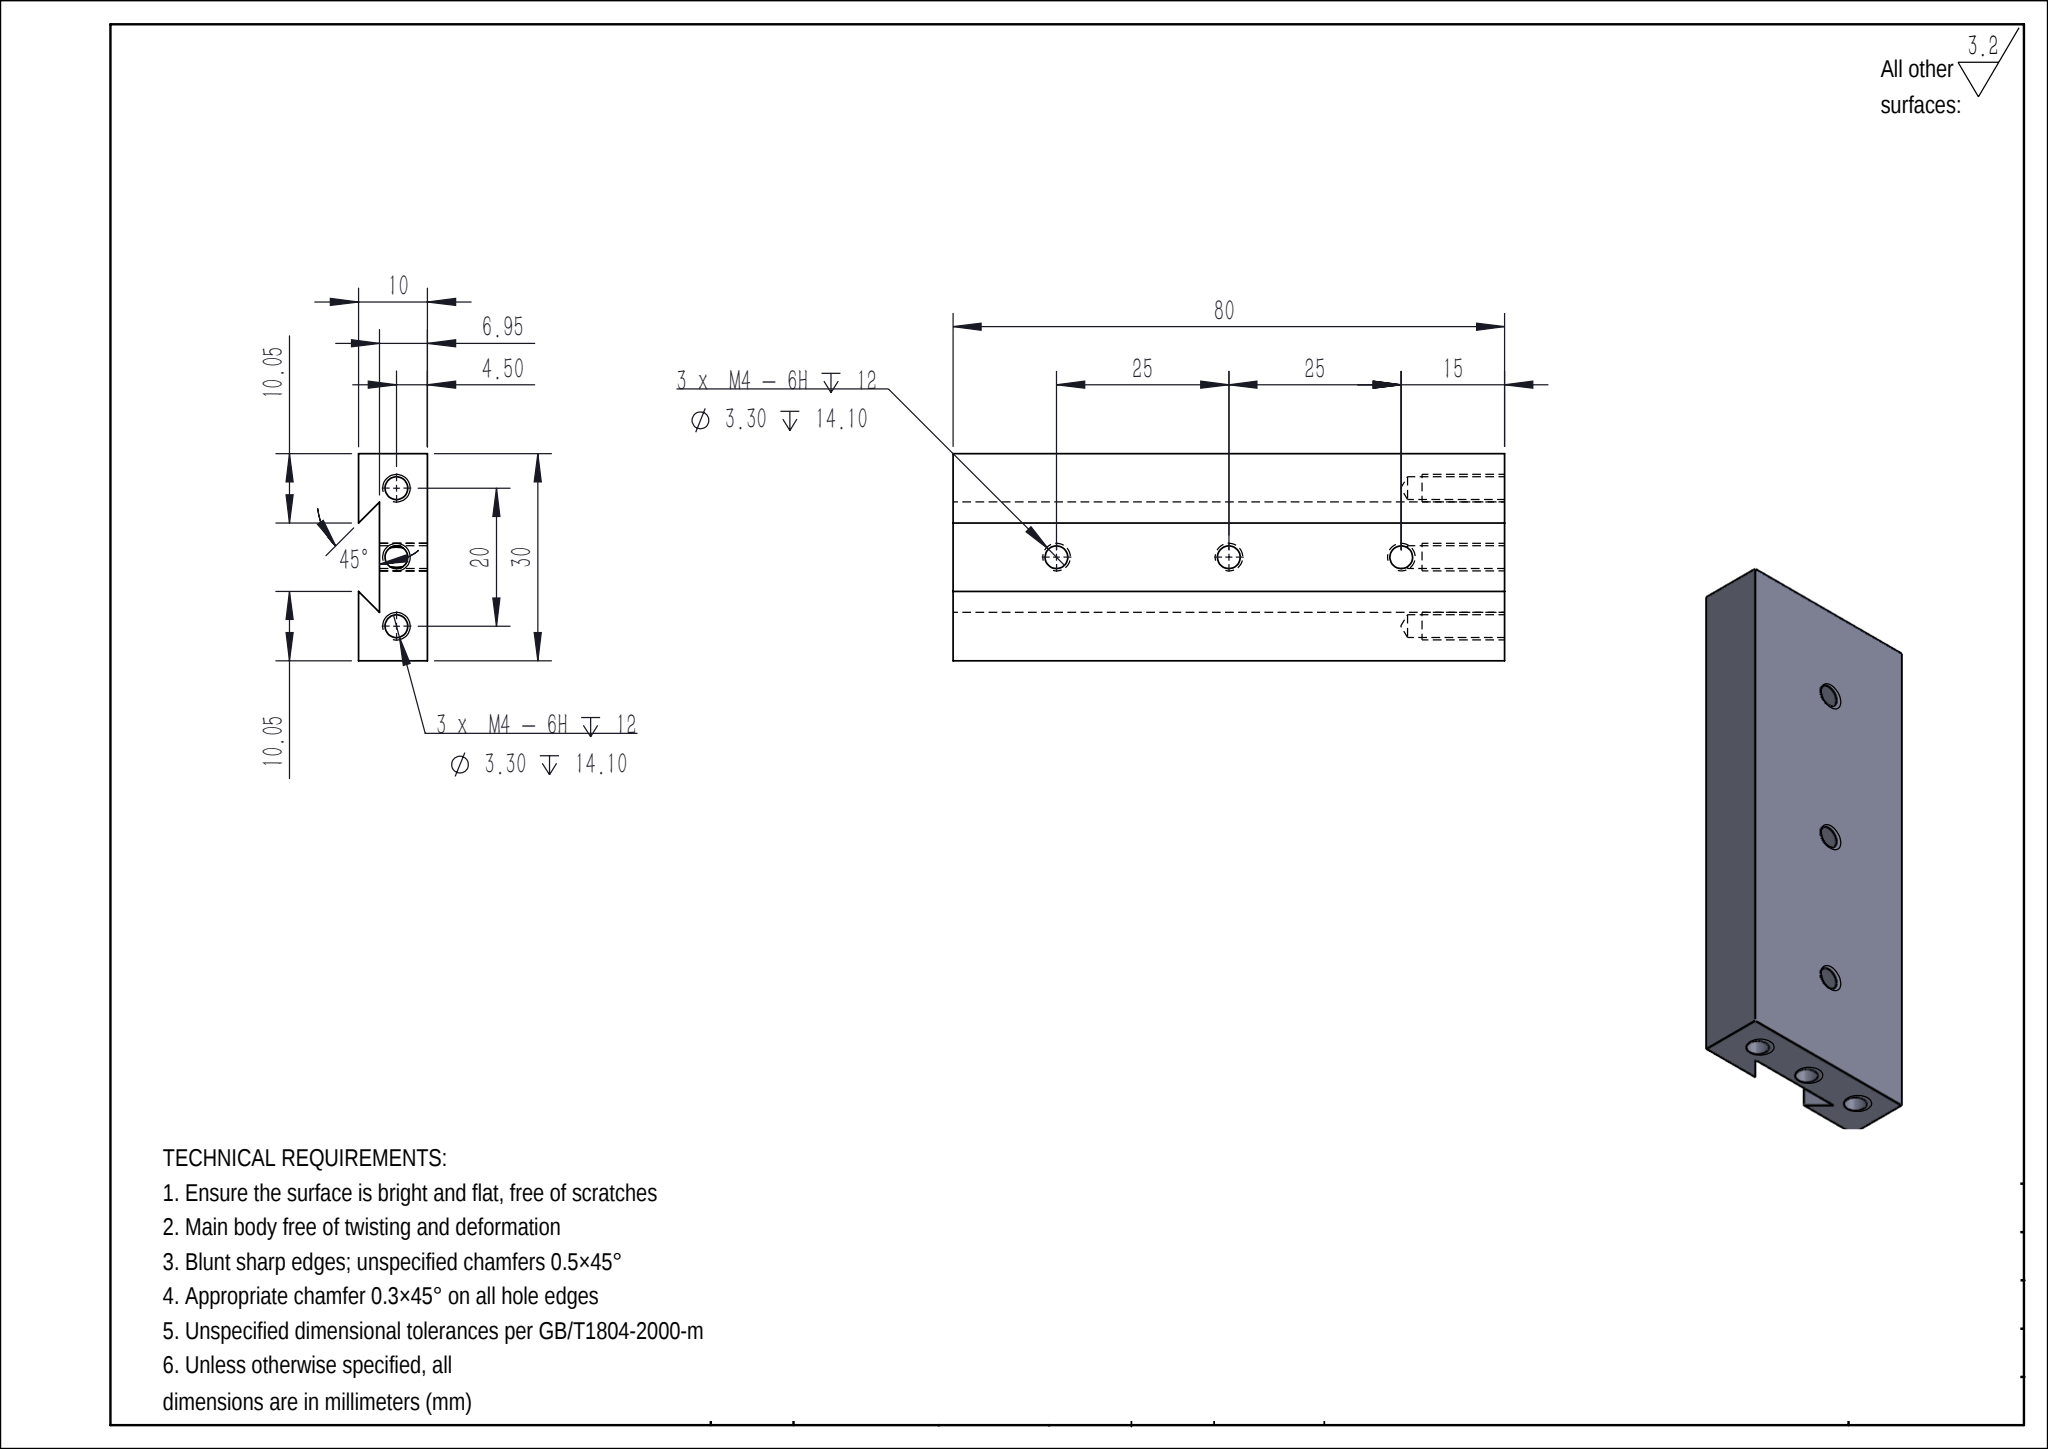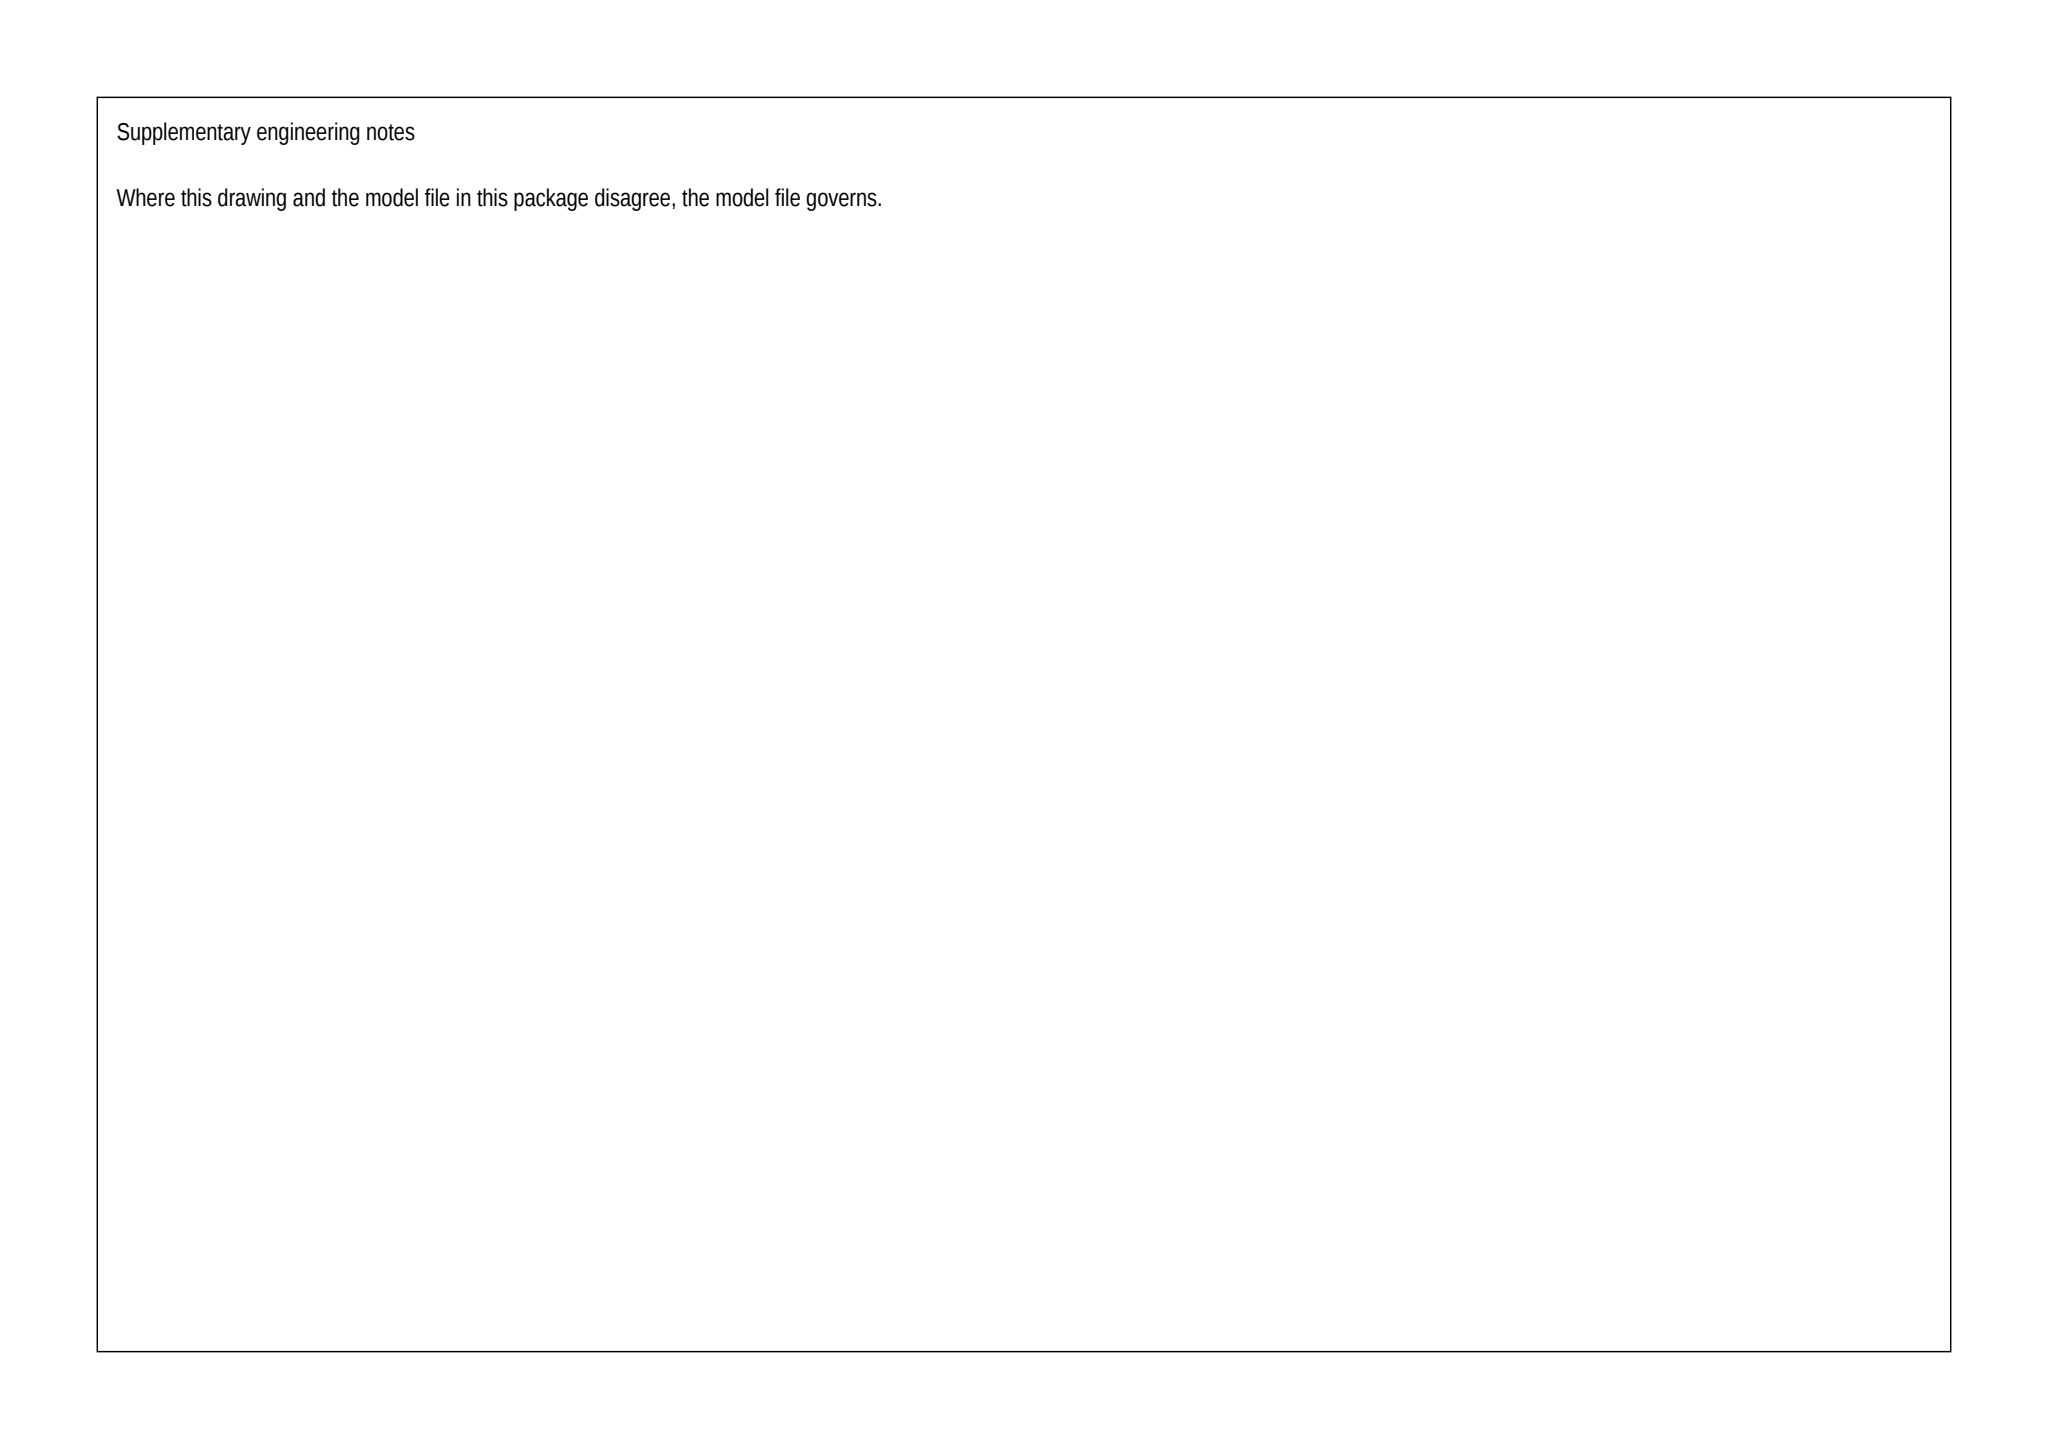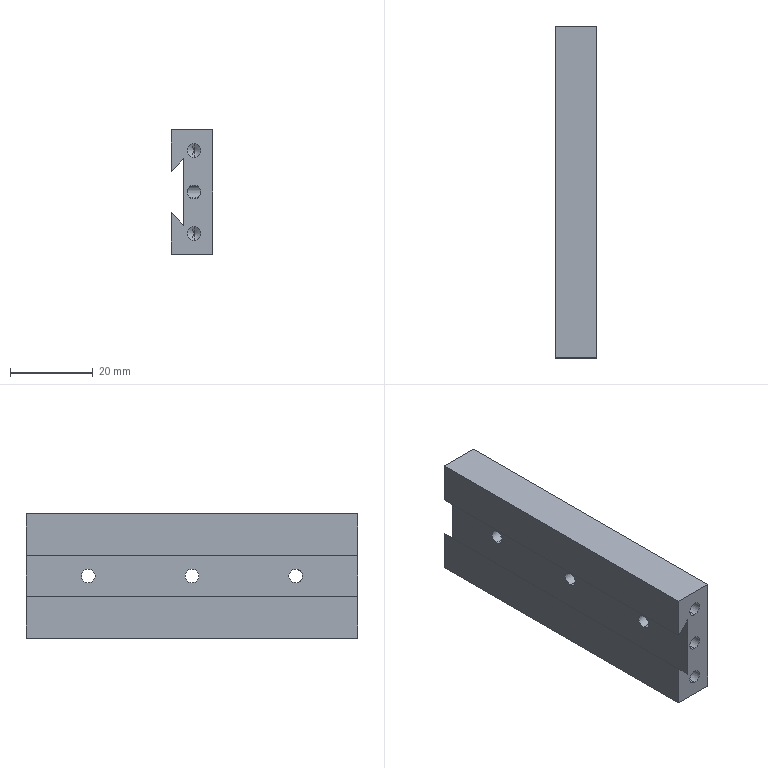Part | SolidWorks | mm | 1 solid | 29 faces | box 10 x 80 x 30 mm | volume 20299 mm3 | cylinder 12 | plane 10 | cone 7 | commonest cylinder face diameters 3.3 x12
build123d program:
from build123d import *

# Parameters (mm, degrees)
SKETCH1_W             = 10
SKETCH1_H             = 80
EXTRUDE_THIN1_DEPTH   = 30
CUT_EXTRUDE1_DEPTH    = 100
M4_TAPPED_HOLE1_D     = 3.3
M4_TAPPED_HOLE1_DEPTH = 14.1
M4_TAPPED_HOLE1_TIP   = 0.9914
M4_TAPPED_HOLE2_D     = 3.3
M4_TAPPED_HOLE2_DEPTH = 14.1
M4_TAPPED_HOLE2_TIP   = 0.9914


with BuildPart() as part:
    # Sketch1 → Extrude-Thin1 (new body)
    with BuildSketch(Plane.XY):
        with Locations((5, 40)):
            Rectangle(SKETCH1_W, SKETCH1_H)
    extrude(amount=EXTRUDE_THIN1_DEPTH)

    # Sketch2 → Cut-Extrude1 (cut)
    with BuildSketch(Plane(origin=(0, 80, 0), x_dir=(1, 0, 0), z_dir=(0, 1, 0))):
        Polygon((0, -10.05), (0, -19.95), (3.05, -23), (3.05, -7), align=None)
    extrude(amount=-CUT_EXTRUDE1_DEPTH, mode=Mode.SUBTRACT)

    # M4 Tapped Hole1
    with Locations(Plane(origin=(0, 0, 0), x_dir=(-1, 0, 0), z_dir=(0, -1, 0))):
        with Locations((-5.5, -5), (-5.5, -25), (-5.5, -15)):
            Hole(M4_TAPPED_HOLE1_D / 2, depth=M4_TAPPED_HOLE1_DEPTH)
            with Locations((0, 0, -(M4_TAPPED_HOLE1_DEPTH + M4_TAPPED_HOLE1_TIP / 2))):  # 118° drill point
                Cone(0, M4_TAPPED_HOLE1_D / 2, M4_TAPPED_HOLE1_TIP, mode=Mode.SUBTRACT)

    # M4 Tapped Hole2
    with Locations(Plane(origin=(10, 0, 0), x_dir=(0, 0, -1), z_dir=(1, 0, 0))):
        with Locations((-15, 40), (-15, 15), (-15, 65)):
            Hole(M4_TAPPED_HOLE2_D / 2, depth=M4_TAPPED_HOLE2_DEPTH)
            with Locations((0, 0, -(M4_TAPPED_HOLE2_DEPTH + M4_TAPPED_HOLE2_TIP / 2))):  # 118° drill point
                Cone(0, M4_TAPPED_HOLE2_D / 2, M4_TAPPED_HOLE2_TIP, mode=Mode.SUBTRACT)


solid = part.part
STEP:
#1=CARTESIAN_POINT('',(3.05,40.,16.65));
#2=VERTEX_POINT('',#1);
#3=CARTESIAN_POINT('',(3.05,40.,13.35));
#4=VERTEX_POINT('',#3);
#5=CARTESIAN_POINT('',(3.05,40.,15.));
#6=DIRECTION('',(1.,0.,0.));
#7=DIRECTION('',(0.,0.,-1.));
#8=AXIS2_PLACEMENT_3D('',#5,#6,#7);
#9=CIRCLE('',#8,1.65);
#10=EDGE_CURVE('',#2,#4,#9,.T.);
#11=ORIENTED_EDGE('',*,*,#10,.F.);
#12=CARTESIAN_POINT('',(10.,40.,16.65));
#13=VERTEX_POINT('',#12);
#14=CARTESIAN_POINT('',(10.,40.,16.65));
#15=DIRECTION('',(1.,0.,0.));
#16=VECTOR('',#15,1000.);
#17=LINE('',#14,#16);
#18=EDGE_CURVE('',#2,#13,#17,.T.);
#19=ORIENTED_EDGE('',*,*,#18,.T.);
#20=CARTESIAN_POINT('',(10.,40.,13.35));
#21=VERTEX_POINT('',#20);
#22=CARTESIAN_POINT('',(10.,40.,15.));
#23=DIRECTION('',(1.,0.,0.));
#24=DIRECTION('',(0.,0.,-1.));
#25=AXIS2_PLACEMENT_3D('',#22,#23,#24);
#26=CIRCLE('',#25,1.65);
#27=EDGE_CURVE('',#13,#21,#26,.T.);
#28=ORIENTED_EDGE('',*,*,#27,.T.);
#29=CARTESIAN_POINT('',(10.,40.,13.35));
#30=DIRECTION('',(1.,0.,0.));
#31=VECTOR('',#30,1000.);
#32=LINE('',#29,#31);
#33=EDGE_CURVE('',#4,#21,#32,.T.);
#34=ORIENTED_EDGE('',*,*,#33,.F.);
#35=EDGE_LOOP('',(#11,#19,#28,#34));
#36=FACE_OUTER_BOUND('',#35,.T.);
#37=CARTESIAN_POINT('',(10.,40.,15.));
#38=DIRECTION('',(1.,0.,0.));
#39=DIRECTION('',(0.,0.,-1.));
#40=AXIS2_PLACEMENT_3D('',#37,#38,#39);
#41=CYLINDRICAL_SURFACE('',#40,1.65);
#42=ADVANCED_FACE('',(#36),#41,.F.);
#43=CARTESIAN_POINT('',(6.4,14.1,16.383));
#44=VERTEX_POINT('',#43);
#45=CARTESIAN_POINT('',(6.4,14.1,13.617));
#46=VERTEX_POINT('',#45);
#47=CARTESIAN_POINT('',(6.4,14.1,16.383));
#48=CARTESIAN_POINT('',(7.509,12.991,15.661));
#49=CARTESIAN_POINT('',(7.509,12.991,14.339));
#50=CARTESIAN_POINT('',(6.4,14.1,13.617));
#51=(BOUNDED_CURVE()B_SPLINE_CURVE(3,(#47,#48,#49,#50),.UNSPECIFIED.,.F.,.F.)B_SPLINE_CURVE_WITH_KNOTS((4,4),(5.289,7.277),.UNSPECIFIED.)CURVE()GEOMETRIC_REPRESENTATION_ITEM()RATIONAL_B_SPLINE_CURVE((1.,0.697,0.697,1.))REPRESENTATION_ITEM(''));
#52=EDGE_CURVE('',#44,#46,#51,.T.);
#53=ORIENTED_EDGE('',*,*,#52,.F.);
#54=CARTESIAN_POINT('',(4.6,14.1,16.383));
#55=VERTEX_POINT('',#54);
#56=CARTESIAN_POINT('',(4.6,14.1,16.383));
#57=CARTESIAN_POINT('',(4.892,14.172,16.43));
#58=CARTESIAN_POINT('',(5.193,14.218,16.453));
#59=CARTESIAN_POINT('',(5.808,14.218,16.453));
#60=CARTESIAN_POINT('',(6.107,14.172,16.43));
#61=CARTESIAN_POINT('',(6.4,14.1,16.383));
#62=B_SPLINE_CURVE_WITH_KNOTS('',3,(#56,#57,#58,#59,#60,#61),.UNSPECIFIED.,.F.,.F.,(4,2,4),(0.0003713,0.001281,0.002191),.UNSPECIFIED.);
#63=EDGE_CURVE('',#55,#44,#62,.T.);
#64=ORIENTED_EDGE('',*,*,#63,.F.);
#65=CARTESIAN_POINT('',(4.6,14.1,13.617));
#66=VERTEX_POINT('',#65);
#67=CARTESIAN_POINT('',(4.6,14.1,13.617));
#68=CARTESIAN_POINT('',(3.491,12.991,14.339));
#69=CARTESIAN_POINT('',(3.491,12.991,15.661));
#70=CARTESIAN_POINT('',(4.6,14.1,16.383));
#71=(BOUNDED_CURVE()B_SPLINE_CURVE(3,(#67,#68,#69,#70),.UNSPECIFIED.,.F.,.F.)B_SPLINE_CURVE_WITH_KNOTS((4,4),(5.289,7.277),.UNSPECIFIED.)CURVE()GEOMETRIC_REPRESENTATION_ITEM()RATIONAL_B_SPLINE_CURVE((1.,0.697,0.697,1.))REPRESENTATION_ITEM(''));
#72=EDGE_CURVE('',#66,#55,#71,.T.);
#73=ORIENTED_EDGE('',*,*,#72,.F.);
#74=CARTESIAN_POINT('',(5.5,14.218,13.547));
#75=VERTEX_POINT('',#74);
#76=CARTESIAN_POINT('',(5.5,14.218,13.547));
#77=CARTESIAN_POINT('',(5.192,14.218,13.547));
#78=CARTESIAN_POINT('',(4.893,14.172,13.57));
#79=CARTESIAN_POINT('',(4.6,14.1,13.617));
#80=B_SPLINE_CURVE_WITH_KNOTS('',3,(#76,#77,#78,#79),.UNSPECIFIED.,.F.,.F.,(4,4),(0.00128,0.002191),.UNSPECIFIED.);
#81=EDGE_CURVE('',#75,#66,#80,.T.);
#82=ORIENTED_EDGE('',*,*,#81,.F.);
#83=CARTESIAN_POINT('',(6.4,14.1,13.617));
#84=CARTESIAN_POINT('',(6.109,14.172,13.57));
#85=CARTESIAN_POINT('',(5.807,14.218,13.547));
#86=CARTESIAN_POINT('',(5.5,14.218,13.547));
#87=B_SPLINE_CURVE_WITH_KNOTS('',3,(#83,#84,#85,#86),.UNSPECIFIED.,.F.,.F.,(4,4),(0.0003713,0.00128),.UNSPECIFIED.);
#88=EDGE_CURVE('',#46,#75,#87,.T.);
#89=ORIENTED_EDGE('',*,*,#88,.F.);
#90=EDGE_LOOP('',(#53,#64,#73,#82,#89));
#91=FACE_BOUND('',#90,.T.);
#92=CARTESIAN_POINT('',(3.05,15.,16.65));
#93=VERTEX_POINT('',#92);
#94=CARTESIAN_POINT('',(3.05,15.,13.35));
#95=VERTEX_POINT('',#94);
#96=CARTESIAN_POINT('',(3.05,15.,15.));
#97=DIRECTION('',(1.,0.,0.));
#98=DIRECTION('',(0.,0.,-1.));
#99=AXIS2_PLACEMENT_3D('',#96,#97,#98);
#100=CIRCLE('',#99,1.65);
#101=EDGE_CURVE('',#93,#95,#100,.T.);
#102=ORIENTED_EDGE('',*,*,#101,.F.);
#103=CARTESIAN_POINT('',(10.,15.,16.65));
#104=VERTEX_POINT('',#103);
#105=CARTESIAN_POINT('',(10.,15.,16.65));
#106=DIRECTION('',(1.,0.,0.));
#107=VECTOR('',#106,1000.);
#108=LINE('',#105,#107);
#109=EDGE_CURVE('',#93,#104,#108,.T.);
#110=ORIENTED_EDGE('',*,*,#109,.T.);
#111=CARTESIAN_POINT('',(10.,15.,13.35));
#112=VERTEX_POINT('',#111);
#113=CARTESIAN_POINT('',(10.,15.,15.));
#114=DIRECTION('',(1.,0.,0.));
#115=DIRECTION('',(0.,0.,-1.));
#116=AXIS2_PLACEMENT_3D('',#113,#114,#115);
#117=CIRCLE('',#116,1.65);
#118=EDGE_CURVE('',#104,#112,#117,.T.);
#119=ORIENTED_EDGE('',*,*,#118,.T.);
#120=CARTESIAN_POINT('',(10.,15.,13.35));
#121=DIRECTION('',(1.,0.,0.));
#122=VECTOR('',#121,1000.);
#123=LINE('',#120,#122);
#124=EDGE_CURVE('',#95,#112,#123,.T.);
#125=ORIENTED_EDGE('',*,*,#124,.F.);
#126=EDGE_LOOP('',(#102,#110,#119,#125));
#127=FACE_OUTER_BOUND('',#126,.T.);
#128=CARTESIAN_POINT('',(10.,15.,15.));
#129=DIRECTION('',(1.,0.,0.));
#130=DIRECTION('',(0.,0.,-1.));
#131=AXIS2_PLACEMENT_3D('',#128,#129,#130);
#132=CYLINDRICAL_SURFACE('',#131,1.65);
#133=ADVANCED_FACE('',(#91,#127),#132,.F.);
#134=CARTESIAN_POINT('',(3.05,65.,16.65));
#135=VERTEX_POINT('',#134);
#136=CARTESIAN_POINT('',(3.05,65.,13.35));
#137=VERTEX_POINT('',#136);
#138=CARTESIAN_POINT('',(3.05,65.,15.));
#139=DIRECTION('',(1.,0.,0.));
#140=DIRECTION('',(0.,0.,-1.));
#141=AXIS2_PLACEMENT_3D('',#138,#139,#140);
#142=CIRCLE('',#141,1.65);
#143=EDGE_CURVE('',#135,#137,#142,.T.);
#144=ORIENTED_EDGE('',*,*,#143,.F.);
#145=CARTESIAN_POINT('',(10.,65.,16.65));
#146=VERTEX_POINT('',#145);
#147=CARTESIAN_POINT('',(10.,65.,16.65));
#148=DIRECTION('',(1.,0.,0.));
#149=VECTOR('',#148,1000.);
#150=LINE('',#147,#149);
#151=EDGE_CURVE('',#135,#146,#150,.T.);
#152=ORIENTED_EDGE('',*,*,#151,.T.);
#153=CARTESIAN_POINT('',(10.,65.,13.35));
#154=VERTEX_POINT('',#153);
#155=CARTESIAN_POINT('',(10.,65.,15.));
#156=DIRECTION('',(1.,0.,0.));
#157=DIRECTION('',(0.,0.,-1.));
#158=AXIS2_PLACEMENT_3D('',#155,#156,#157);
#159=CIRCLE('',#158,1.65);
#160=EDGE_CURVE('',#146,#154,#159,.T.);
#161=ORIENTED_EDGE('',*,*,#160,.T.);
#162=CARTESIAN_POINT('',(10.,65.,13.35));
#163=DIRECTION('',(1.,0.,0.));
#164=VECTOR('',#163,1000.);
#165=LINE('',#162,#164);
#166=EDGE_CURVE('',#137,#154,#165,.T.);
#167=ORIENTED_EDGE('',*,*,#166,.F.);
#168=EDGE_LOOP('',(#144,#152,#161,#167));
#169=FACE_OUTER_BOUND('',#168,.T.);
#170=CARTESIAN_POINT('',(10.,65.,15.));
#171=DIRECTION('',(1.,0.,0.));
#172=DIRECTION('',(0.,0.,-1.));
#173=AXIS2_PLACEMENT_3D('',#170,#171,#172);
#174=CYLINDRICAL_SURFACE('',#173,1.65);
#175=ADVANCED_FACE('',(#169),#174,.F.);
#176=CARTESIAN_POINT('',(5.5,14.1,6.65));
#177=VERTEX_POINT('',#176);
#178=CARTESIAN_POINT('',(5.5,14.1,3.35));
#179=VERTEX_POINT('',#178);
#180=CARTESIAN_POINT('',(5.5,14.1,5.));
#181=DIRECTION('',(0.,-1.,0.));
#182=DIRECTION('',(0.,0.,-1.));
#183=AXIS2_PLACEMENT_3D('',#180,#181,#182);
#184=CIRCLE('',#183,1.65);
#185=EDGE_CURVE('',#177,#179,#184,.T.);
#186=ORIENTED_EDGE('',*,*,#185,.F.);
#187=CARTESIAN_POINT('',(5.5,-0.,6.65));
#188=VERTEX_POINT('',#187);
#189=CARTESIAN_POINT('',(5.5,0.,6.65));
#190=DIRECTION('',(0.,-1.,0.));
#191=VECTOR('',#190,1000.);
#192=LINE('',#189,#191);
#193=EDGE_CURVE('',#177,#188,#192,.T.);
#194=ORIENTED_EDGE('',*,*,#193,.T.);
#195=CARTESIAN_POINT('',(5.5,-0.,3.35));
#196=VERTEX_POINT('',#195);
#197=CARTESIAN_POINT('',(5.5,-0.,5.));
#198=DIRECTION('',(0.,-1.,0.));
#199=DIRECTION('',(0.,0.,-1.));
#200=AXIS2_PLACEMENT_3D('',#197,#198,#199);
#201=CIRCLE('',#200,1.65);
#202=EDGE_CURVE('',#188,#196,#201,.T.);
#203=ORIENTED_EDGE('',*,*,#202,.T.);
#204=CARTESIAN_POINT('',(5.5,0.,3.35));
#205=DIRECTION('',(0.,-1.,0.));
#206=VECTOR('',#205,1000.);
#207=LINE('',#204,#206);
#208=EDGE_CURVE('',#179,#196,#207,.T.);
#209=ORIENTED_EDGE('',*,*,#208,.F.);
#210=EDGE_LOOP('',(#186,#194,#203,#209));
#211=FACE_OUTER_BOUND('',#210,.T.);
#212=CARTESIAN_POINT('',(5.5,0.,5.));
#213=DIRECTION('',(0.,-1.,0.));
#214=DIRECTION('',(0.,0.,-1.));
#215=AXIS2_PLACEMENT_3D('',#212,#213,#214);
#216=CYLINDRICAL_SURFACE('',#215,1.65);
#217=ADVANCED_FACE('',(#211),#216,.F.);
#218=CARTESIAN_POINT('',(5.5,15.091,5.));
#219=VERTEX_POINT('',#218);
#220=CARTESIAN_POINT('',(5.5,14.1,3.35));
#221=DIRECTION('',(0.,-0.515,-0.8572));
#222=VECTOR('',#221,1000.);
#223=LINE('',#220,#222);
#224=EDGE_CURVE('',#219,#179,#223,.T.);
#225=ORIENTED_EDGE('',*,*,#224,.F.);
#226=CARTESIAN_POINT('',(5.5,14.1,6.65));
#227=DIRECTION('',(0.,-0.515,0.8572));
#228=VECTOR('',#227,1000.);
#229=LINE('',#226,#228);
#230=EDGE_CURVE('',#219,#177,#229,.T.);
#231=ORIENTED_EDGE('',*,*,#230,.T.);
#232=ORIENTED_EDGE('',*,*,#185,.T.);
#233=EDGE_LOOP('',(#225,#231,#232));
#234=FACE_OUTER_BOUND('',#233,.T.);
#235=CARTESIAN_POINT('',(5.5,14.1,5.));
#236=DIRECTION('',(0.,-1.,0.));
#237=DIRECTION('',(0.,0.,-1.));
#238=AXIS2_PLACEMENT_3D('',#235,#236,#237);
#239=CONICAL_SURFACE('',#238,1.65,1.03);
#240=ADVANCED_FACE('',(#234),#239,.F.);
#241=CARTESIAN_POINT('',(5.5,14.1,26.65));
#242=VERTEX_POINT('',#241);
#243=CARTESIAN_POINT('',(5.5,14.1,23.35));
#244=VERTEX_POINT('',#243);
#245=CARTESIAN_POINT('',(5.5,14.1,25.));
#246=DIRECTION('',(0.,-1.,0.));
#247=DIRECTION('',(0.,0.,-1.));
#248=AXIS2_PLACEMENT_3D('',#245,#246,#247);
#249=CIRCLE('',#248,1.65);
#250=EDGE_CURVE('',#242,#244,#249,.T.);
#251=ORIENTED_EDGE('',*,*,#250,.F.);
#252=CARTESIAN_POINT('',(5.5,-0.,26.65));
#253=VERTEX_POINT('',#252);
#254=CARTESIAN_POINT('',(5.5,0.,26.65));
#255=DIRECTION('',(0.,-1.,0.));
#256=VECTOR('',#255,1000.);
#257=LINE('',#254,#256);
#258=EDGE_CURVE('',#242,#253,#257,.T.);
#259=ORIENTED_EDGE('',*,*,#258,.T.);
#260=CARTESIAN_POINT('',(5.5,-0.,23.35));
#261=VERTEX_POINT('',#260);
#262=CARTESIAN_POINT('',(5.5,-0.,25.));
#263=DIRECTION('',(0.,-1.,0.));
#264=DIRECTION('',(0.,0.,-1.));
#265=AXIS2_PLACEMENT_3D('',#262,#263,#264);
#266=CIRCLE('',#265,1.65);
#267=EDGE_CURVE('',#253,#261,#266,.T.);
#268=ORIENTED_EDGE('',*,*,#267,.T.);
#269=CARTESIAN_POINT('',(5.5,0.,23.35));
#270=DIRECTION('',(0.,-1.,0.));
#271=VECTOR('',#270,1000.);
#272=LINE('',#269,#271);
#273=EDGE_CURVE('',#244,#261,#272,.T.);
#274=ORIENTED_EDGE('',*,*,#273,.F.);
#275=EDGE_LOOP('',(#251,#259,#268,#274));
#276=FACE_OUTER_BOUND('',#275,.T.);
#277=CARTESIAN_POINT('',(5.5,0.,25.));
#278=DIRECTION('',(0.,-1.,0.));
#279=DIRECTION('',(0.,0.,-1.));
#280=AXIS2_PLACEMENT_3D('',#277,#278,#279);
#281=CYLINDRICAL_SURFACE('',#280,1.65);
#282=ADVANCED_FACE('',(#276),#281,.F.);
#283=CARTESIAN_POINT('',(5.5,15.091,25.));
#284=VERTEX_POINT('',#283);
#285=CARTESIAN_POINT('',(5.5,14.1,23.35));
#286=DIRECTION('',(0.,-0.515,-0.8572));
#287=VECTOR('',#286,1000.);
#288=LINE('',#285,#287);
#289=EDGE_CURVE('',#284,#244,#288,.T.);
#290=ORIENTED_EDGE('',*,*,#289,.F.);
#291=CARTESIAN_POINT('',(5.5,14.1,26.65));
#292=DIRECTION('',(0.,-0.515,0.8572));
#293=VECTOR('',#292,1000.);
#294=LINE('',#291,#293);
#295=EDGE_CURVE('',#284,#242,#294,.T.);
#296=ORIENTED_EDGE('',*,*,#295,.T.);
#297=ORIENTED_EDGE('',*,*,#250,.T.);
#298=EDGE_LOOP('',(#290,#296,#297));
#299=FACE_OUTER_BOUND('',#298,.T.);
#300=CARTESIAN_POINT('',(5.5,14.1,25.));
#301=DIRECTION('',(0.,-1.,0.));
#302=DIRECTION('',(0.,0.,-1.));
#303=AXIS2_PLACEMENT_3D('',#300,#301,#302);
#304=CONICAL_SURFACE('',#303,1.65,1.03);
#305=ADVANCED_FACE('',(#299),#304,.F.);
#306=CARTESIAN_POINT('',(5.5,14.1,16.65));
#307=VERTEX_POINT('',#306);
#308=CARTESIAN_POINT('',(5.5,14.1,15.));
#309=DIRECTION('',(0.,-1.,0.));
#310=DIRECTION('',(0.,0.,-1.));
#311=AXIS2_PLACEMENT_3D('',#308,#309,#310);
#312=CIRCLE('',#311,1.65);
#313=EDGE_CURVE('',#307,#55,#312,.T.);
#314=ORIENTED_EDGE('',*,*,#313,.F.);
#315=CARTESIAN_POINT('',(5.5,-0.,16.65));
#316=VERTEX_POINT('',#315);
#317=CARTESIAN_POINT('',(5.5,0.,16.65));
#318=DIRECTION('',(0.,-1.,0.));
#319=VECTOR('',#318,1000.);
#320=LINE('',#317,#319);
#321=EDGE_CURVE('',#307,#316,#320,.T.);
#322=ORIENTED_EDGE('',*,*,#321,.T.);
#323=CARTESIAN_POINT('',(5.5,-0.,13.35));
#324=VERTEX_POINT('',#323);
#325=CARTESIAN_POINT('',(5.5,-0.,15.));
#326=DIRECTION('',(0.,-1.,0.));
#327=DIRECTION('',(0.,0.,-1.));
#328=AXIS2_PLACEMENT_3D('',#325,#326,#327);
#329=CIRCLE('',#328,1.65);
#330=EDGE_CURVE('',#316,#324,#329,.T.);
#331=ORIENTED_EDGE('',*,*,#330,.T.);
#332=CARTESIAN_POINT('',(5.5,14.1,13.35));
#333=VERTEX_POINT('',#332);
#334=CARTESIAN_POINT('',(5.5,0.,13.35));
#335=DIRECTION('',(0.,-1.,0.));
#336=VECTOR('',#335,1000.);
#337=LINE('',#334,#336);
#338=EDGE_CURVE('',#333,#324,#337,.T.);
#339=ORIENTED_EDGE('',*,*,#338,.F.);
#340=CARTESIAN_POINT('',(5.5,14.1,15.));
#341=DIRECTION('',(0.,-1.,0.));
#342=DIRECTION('',(0.,0.,-1.));
#343=AXIS2_PLACEMENT_3D('',#340,#341,#342);
#344=CIRCLE('',#343,1.65);
#345=EDGE_CURVE('',#66,#333,#344,.T.);
#346=ORIENTED_EDGE('',*,*,#345,.F.);
#347=ORIENTED_EDGE('',*,*,#72,.T.);
#348=EDGE_LOOP('',(#314,#322,#331,#339,#346,#347));
#349=FACE_OUTER_BOUND('',#348,.T.);
#350=CARTESIAN_POINT('',(5.5,0.,15.));
#351=DIRECTION('',(0.,-1.,0.));
#352=DIRECTION('',(0.,0.,-1.));
#353=AXIS2_PLACEMENT_3D('',#350,#351,#352);
#354=CYLINDRICAL_SURFACE('',#353,1.65);
#355=ADVANCED_FACE('',(#349),#354,.F.);
#356=ORIENTED_EDGE('',*,*,#88,.T.);
#357=CARTESIAN_POINT('',(5.5,14.1,13.35));
#358=DIRECTION('',(0.,-0.515,-0.8572));
#359=VECTOR('',#358,1000.);
#360=LINE('',#357,#359);
#361=EDGE_CURVE('',#75,#333,#360,.T.);
#362=ORIENTED_EDGE('',*,*,#361,.T.);
#363=CARTESIAN_POINT('',(5.5,14.1,15.));
#364=DIRECTION('',(0.,-1.,0.));
#365=DIRECTION('',(0.,0.,-1.));
#366=AXIS2_PLACEMENT_3D('',#363,#364,#365);
#367=CIRCLE('',#366,1.65);
#368=EDGE_CURVE('',#333,#46,#367,.T.);
#369=ORIENTED_EDGE('',*,*,#368,.T.);
#370=EDGE_LOOP('',(#356,#362,#369));
#371=FACE_OUTER_BOUND('',#370,.T.);
#372=CARTESIAN_POINT('',(5.5,14.1,15.));
#373=DIRECTION('',(0.,-1.,0.));
#374=DIRECTION('',(0.,0.,-1.));
#375=AXIS2_PLACEMENT_3D('',#372,#373,#374);
#376=CONICAL_SURFACE('',#375,1.65,1.03);
#377=ADVANCED_FACE('',(#371),#376,.F.);
#378=ORIENTED_EDGE('',*,*,#361,.F.);
#379=ORIENTED_EDGE('',*,*,#81,.T.);
#380=ORIENTED_EDGE('',*,*,#345,.T.);
#381=EDGE_LOOP('',(#378,#379,#380));
#382=FACE_OUTER_BOUND('',#381,.T.);
#383=CARTESIAN_POINT('',(5.5,14.1,15.));
#384=DIRECTION('',(0.,-1.,0.));
#385=DIRECTION('',(0.,0.,-1.));
#386=AXIS2_PLACEMENT_3D('',#383,#384,#385);
#387=CONICAL_SURFACE('',#386,1.65,1.03);
#388=ADVANCED_FACE('',(#382),#387,.F.);
#389=CARTESIAN_POINT('',(-0.,0.,10.05));
#390=VERTEX_POINT('',#389);
#391=CARTESIAN_POINT('',(-0.,80.,10.05));
#392=VERTEX_POINT('',#391);
#393=CARTESIAN_POINT('',(-0.,-20.,10.05));
#394=DIRECTION('',(0.,1.,0.));
#395=VECTOR('',#394,1000.);
#396=LINE('',#393,#395);
#397=EDGE_CURVE('',#390,#392,#396,.T.);
#398=ORIENTED_EDGE('',*,*,#397,.T.);
#399=CARTESIAN_POINT('',(0.,80.,0.));
#400=VERTEX_POINT('',#399);
#401=CARTESIAN_POINT('',(0.,80.,30.));
#402=DIRECTION('',(0.,0.,-1.));
#403=VECTOR('',#402,1000.);
#404=LINE('',#401,#403);
#405=EDGE_CURVE('',#392,#400,#404,.T.);
#406=ORIENTED_EDGE('',*,*,#405,.T.);
#407=CARTESIAN_POINT('',(0.,0.,0.));
#408=VERTEX_POINT('',#407);
#409=CARTESIAN_POINT('',(0.,0.,0.));
#410=DIRECTION('',(0.,1.,0.));
#411=VECTOR('',#410,1000.);
#412=LINE('',#409,#411);
#413=EDGE_CURVE('',#408,#400,#412,.T.);
#414=ORIENTED_EDGE('',*,*,#413,.F.);
#415=CARTESIAN_POINT('',(0.,0.,30.));
#416=DIRECTION('',(0.,0.,-1.));
#417=VECTOR('',#416,1000.);
#418=LINE('',#415,#417);
#419=EDGE_CURVE('',#390,#408,#418,.T.);
#420=ORIENTED_EDGE('',*,*,#419,.F.);
#421=EDGE_LOOP('',(#398,#406,#414,#420));
#422=FACE_OUTER_BOUND('',#421,.T.);
#423=CARTESIAN_POINT('',(0.,0.,30.));
#424=DIRECTION('',(-1.,0.,0.));
#425=DIRECTION('',(0.,0.,1.));
#426=AXIS2_PLACEMENT_3D('',#423,#424,#425);
#427=PLANE('',#426);
#428=ADVANCED_FACE('',(#422),#427,.T.);
#429=CARTESIAN_POINT('',(10.,40.,15.));
#430=DIRECTION('',(1.,0.,0.));
#431=DIRECTION('',(0.,0.,-1.));
#432=AXIS2_PLACEMENT_3D('',#429,#430,#431);
#433=CIRCLE('',#432,1.65);
#434=EDGE_CURVE('',#21,#13,#433,.T.);
#435=ORIENTED_EDGE('',*,*,#434,.F.);
#436=ORIENTED_EDGE('',*,*,#27,.F.);
#437=EDGE_LOOP('',(#435,#436));
#438=FACE_BOUND('',#437,.T.);
#439=CARTESIAN_POINT('',(10.,15.,15.));
#440=DIRECTION('',(1.,0.,0.));
#441=DIRECTION('',(0.,0.,-1.));
#442=AXIS2_PLACEMENT_3D('',#439,#440,#441);
#443=CIRCLE('',#442,1.65);
#444=EDGE_CURVE('',#112,#104,#443,.T.);
#445=ORIENTED_EDGE('',*,*,#444,.F.);
#446=ORIENTED_EDGE('',*,*,#118,.F.);
#447=EDGE_LOOP('',(#445,#446));
#448=FACE_BOUND('',#447,.T.);
#449=CARTESIAN_POINT('',(10.,65.,15.));
#450=DIRECTION('',(1.,0.,0.));
#451=DIRECTION('',(0.,0.,-1.));
#452=AXIS2_PLACEMENT_3D('',#449,#450,#451);
#453=CIRCLE('',#452,1.65);
#454=EDGE_CURVE('',#154,#146,#453,.T.);
#455=ORIENTED_EDGE('',*,*,#454,.F.);
#456=ORIENTED_EDGE('',*,*,#160,.F.);
#457=EDGE_LOOP('',(#455,#456));
#458=FACE_BOUND('',#457,.T.);
#459=CARTESIAN_POINT('',(10.,0.,0.));
#460=VERTEX_POINT('',#459);
#461=CARTESIAN_POINT('',(10.,80.,0.));
#462=VERTEX_POINT('',#461);
#463=CARTESIAN_POINT('',(10.,0.,0.));
#464=DIRECTION('',(0.,1.,0.));
#465=VECTOR('',#464,1000.);
#466=LINE('',#463,#465);
#467=EDGE_CURVE('',#460,#462,#466,.T.);
#468=ORIENTED_EDGE('',*,*,#467,.T.);
#469=CARTESIAN_POINT('',(10.,80.,30.));
#470=VERTEX_POINT('',#469);
#471=CARTESIAN_POINT('',(10.,80.,30.));
#472=DIRECTION('',(0.,0.,-1.));
#473=VECTOR('',#472,1000.);
#474=LINE('',#471,#473);
#475=EDGE_CURVE('',#470,#462,#474,.T.);
#476=ORIENTED_EDGE('',*,*,#475,.F.);
#477=CARTESIAN_POINT('',(10.,0.,30.));
#478=VERTEX_POINT('',#477);
#479=CARTESIAN_POINT('',(10.,0.,30.));
#480=DIRECTION('',(0.,1.,0.));
#481=VECTOR('',#480,1000.);
#482=LINE('',#479,#481);
#483=EDGE_CURVE('',#478,#470,#482,.T.);
#484=ORIENTED_EDGE('',*,*,#483,.F.);
#485=CARTESIAN_POINT('',(10.,0.,30.));
#486=DIRECTION('',(0.,0.,-1.));
#487=VECTOR('',#486,1000.);
#488=LINE('',#485,#487);
#489=EDGE_CURVE('',#478,#460,#488,.T.);
#490=ORIENTED_EDGE('',*,*,#489,.T.);
#491=EDGE_LOOP('',(#468,#476,#484,#490));
#492=FACE_OUTER_BOUND('',#491,.T.);
#493=CARTESIAN_POINT('',(10.,0.,30.));
#494=DIRECTION('',(-1.,0.,0.));
#495=DIRECTION('',(0.,0.,1.));
#496=AXIS2_PLACEMENT_3D('',#493,#494,#495);
#497=PLANE('',#496);
#498=ADVANCED_FACE('',(#438,#448,#458,#492),#497,.F.);
#499=CARTESIAN_POINT('',(3.05,80.,7.));
#500=VERTEX_POINT('',#499);
#501=CARTESIAN_POINT('',(3.05,80.,7.));
#502=DIRECTION('',(-0.7071,0.,0.7071));
#503=VECTOR('',#502,1000.);
#504=LINE('',#501,#503);
#505=EDGE_CURVE('',#500,#392,#504,.T.);
#506=ORIENTED_EDGE('',*,*,#505,.F.);
#507=CARTESIAN_POINT('',(3.05,80.,23.));
#508=VERTEX_POINT('',#507);
#509=CARTESIAN_POINT('',(3.05,80.,23.));
#510=DIRECTION('',(0.,0.,-1.));
#511=VECTOR('',#510,1000.);
#512=LINE('',#509,#511);
#513=EDGE_CURVE('',#508,#500,#512,.T.);
#514=ORIENTED_EDGE('',*,*,#513,.F.);
#515=CARTESIAN_POINT('',(0.,80.,19.95));
#516=VERTEX_POINT('',#515);
#517=CARTESIAN_POINT('',(0.,80.,19.95));
#518=DIRECTION('',(0.7071,0.,0.7071));
#519=VECTOR('',#518,1000.);
#520=LINE('',#517,#519);
#521=EDGE_CURVE('',#516,#508,#520,.T.);
#522=ORIENTED_EDGE('',*,*,#521,.F.);
#523=CARTESIAN_POINT('',(0.,80.,30.));
#524=VERTEX_POINT('',#523);
#525=CARTESIAN_POINT('',(0.,80.,30.));
#526=DIRECTION('',(0.,0.,-1.));
#527=VECTOR('',#526,1000.);
#528=LINE('',#525,#527);
#529=EDGE_CURVE('',#524,#516,#528,.T.);
#530=ORIENTED_EDGE('',*,*,#529,.F.);
#531=CARTESIAN_POINT('',(0.,80.,30.));
#532=DIRECTION('',(1.,0.,0.));
#533=VECTOR('',#532,1000.);
#534=LINE('',#531,#533);
#535=EDGE_CURVE('',#524,#470,#534,.T.);
#536=ORIENTED_EDGE('',*,*,#535,.T.);
#537=ORIENTED_EDGE('',*,*,#475,.T.);
#538=CARTESIAN_POINT('',(0.,80.,0.));
#539=DIRECTION('',(1.,0.,0.));
#540=VECTOR('',#539,1000.);
#541=LINE('',#538,#540);
#542=EDGE_CURVE('',#400,#462,#541,.T.);
#543=ORIENTED_EDGE('',*,*,#542,.F.);
#544=ORIENTED_EDGE('',*,*,#405,.F.);
#545=EDGE_LOOP('',(#506,#514,#522,#530,#536,#537,#543,#544));
#546=FACE_OUTER_BOUND('',#545,.T.);
#547=CARTESIAN_POINT('',(0.,80.,30.));
#548=DIRECTION('',(0.,1.,0.));
#549=DIRECTION('',(0.,0.,1.));
#550=AXIS2_PLACEMENT_3D('',#547,#548,#549);
#551=PLANE('',#550);
#552=ADVANCED_FACE('',(#546),#551,.T.);
#553=CARTESIAN_POINT('',(0.,0.,19.95));
#554=VERTEX_POINT('',#553);
#555=CARTESIAN_POINT('',(0.,-20.,19.95));
#556=DIRECTION('',(0.,1.,0.));
#557=VECTOR('',#556,1000.);
#558=LINE('',#555,#557);
#559=EDGE_CURVE('',#554,#516,#558,.T.);
#560=ORIENTED_EDGE('',*,*,#559,.F.);
#561=CARTESIAN_POINT('',(0.,0.,30.));
#562=VERTEX_POINT('',#561);
#563=CARTESIAN_POINT('',(0.,0.,30.));
#564=DIRECTION('',(0.,0.,-1.));
#565=VECTOR('',#564,1000.);
#566=LINE('',#563,#565);
#567=EDGE_CURVE('',#562,#554,#566,.T.);
#568=ORIENTED_EDGE('',*,*,#567,.F.);
#569=CARTESIAN_POINT('',(0.,0.,30.));
#570=DIRECTION('',(0.,1.,0.));
#571=VECTOR('',#570,1000.);
#572=LINE('',#569,#571);
#573=EDGE_CURVE('',#562,#524,#572,.T.);
#574=ORIENTED_EDGE('',*,*,#573,.T.);
#575=ORIENTED_EDGE('',*,*,#529,.T.);
#576=EDGE_LOOP('',(#560,#568,#574,#575));
#577=FACE_OUTER_BOUND('',#576,.T.);
#578=CARTESIAN_POINT('',(0.,0.,30.));
#579=DIRECTION('',(-1.,0.,0.));
#580=DIRECTION('',(0.,0.,1.));
#581=AXIS2_PLACEMENT_3D('',#578,#579,#580);
#582=PLANE('',#581);
#583=ADVANCED_FACE('',(#577),#582,.T.);
#584=CARTESIAN_POINT('',(5.5,-0.,5.));
#585=DIRECTION('',(0.,-1.,0.));
#586=DIRECTION('',(0.,0.,-1.));
#587=AXIS2_PLACEMENT_3D('',#584,#585,#586);
#588=CIRCLE('',#587,1.65);
#589=EDGE_CURVE('',#196,#188,#588,.T.);
#590=ORIENTED_EDGE('',*,*,#589,.F.);
#591=ORIENTED_EDGE('',*,*,#202,.F.);
#592=EDGE_LOOP('',(#590,#591));
#593=FACE_BOUND('',#592,.T.);
#594=CARTESIAN_POINT('',(5.5,-0.,25.));
#595=DIRECTION('',(0.,-1.,0.));
#596=DIRECTION('',(0.,0.,-1.));
#597=AXIS2_PLACEMENT_3D('',#594,#595,#596);
#598=CIRCLE('',#597,1.65);
#599=EDGE_CURVE('',#261,#253,#598,.T.);
#600=ORIENTED_EDGE('',*,*,#599,.F.);
#601=ORIENTED_EDGE('',*,*,#267,.F.);
#602=EDGE_LOOP('',(#600,#601));
#603=FACE_BOUND('',#602,.T.);
#604=CARTESIAN_POINT('',(5.5,-0.,15.));
#605=DIRECTION('',(0.,-1.,0.));
#606=DIRECTION('',(0.,0.,-1.));
#607=AXIS2_PLACEMENT_3D('',#604,#605,#606);
#608=CIRCLE('',#607,1.65);
#609=EDGE_CURVE('',#324,#316,#608,.T.);
#610=ORIENTED_EDGE('',*,*,#609,.F.);
#611=ORIENTED_EDGE('',*,*,#330,.F.);
#612=EDGE_LOOP('',(#610,#611));
#613=FACE_BOUND('',#612,.T.);
#614=CARTESIAN_POINT('',(3.05,0.,7.));
#615=VERTEX_POINT('',#614);
#616=CARTESIAN_POINT('',(-4.975,0.,15.025));
#617=DIRECTION('',(0.7071,0.,-0.7071));
#618=VECTOR('',#617,1000.);
#619=LINE('',#616,#618);
#620=EDGE_CURVE('',#390,#615,#619,.T.);
#621=ORIENTED_EDGE('',*,*,#620,.F.);
#622=ORIENTED_EDGE('',*,*,#419,.T.);
#623=CARTESIAN_POINT('',(10.,0.,0.));
#624=DIRECTION('',(-1.,0.,0.));
#625=VECTOR('',#624,1000.);
#626=LINE('',#623,#625);
#627=EDGE_CURVE('',#460,#408,#626,.T.);
#628=ORIENTED_EDGE('',*,*,#627,.F.);
#629=ORIENTED_EDGE('',*,*,#489,.F.);
#630=CARTESIAN_POINT('',(10.,0.,30.));
#631=DIRECTION('',(-1.,0.,0.));
#632=VECTOR('',#631,1000.);
#633=LINE('',#630,#632);
#634=EDGE_CURVE('',#478,#562,#633,.T.);
#635=ORIENTED_EDGE('',*,*,#634,.T.);
#636=ORIENTED_EDGE('',*,*,#567,.T.);
#637=CARTESIAN_POINT('',(3.05,0.,23.));
#638=VERTEX_POINT('',#637);
#639=CARTESIAN_POINT('',(10.025,0.,29.975));
#640=DIRECTION('',(-0.7071,0.,-0.7071));
#641=VECTOR('',#640,1000.);
#642=LINE('',#639,#641);
#643=EDGE_CURVE('',#638,#554,#642,.T.);
#644=ORIENTED_EDGE('',*,*,#643,.F.);
#645=CARTESIAN_POINT('',(3.05,0.,30.));
#646=DIRECTION('',(0.,0.,1.));
#647=VECTOR('',#646,1000.);
#648=LINE('',#645,#647);
#649=EDGE_CURVE('',#615,#638,#648,.T.);
#650=ORIENTED_EDGE('',*,*,#649,.F.);
#651=EDGE_LOOP('',(#621,#622,#628,#629,#635,#636,#644,#650));
#652=FACE_OUTER_BOUND('',#651,.T.);
#653=CARTESIAN_POINT('',(10.,0.,30.));
#654=DIRECTION('',(0.,-1.,0.));
#655=DIRECTION('',(0.,0.,-1.));
#656=AXIS2_PLACEMENT_3D('',#653,#654,#655);
#657=PLANE('',#656);
#658=ADVANCED_FACE('',(#593,#603,#613,#652),#657,.T.);
#659=ORIENTED_EDGE('',*,*,#483,.T.);
#660=ORIENTED_EDGE('',*,*,#535,.F.);
#661=ORIENTED_EDGE('',*,*,#573,.F.);
#662=ORIENTED_EDGE('',*,*,#634,.F.);
#663=EDGE_LOOP('',(#659,#660,#661,#662));
#664=FACE_OUTER_BOUND('',#663,.T.);
#665=CARTESIAN_POINT('',(0.,0.,30.));
#666=DIRECTION('',(0.,0.,-1.));
#667=DIRECTION('',(-1.,0.,0.));
#668=AXIS2_PLACEMENT_3D('',#665,#666,#667);
#669=PLANE('',#668);
#670=ADVANCED_FACE('',(#664),#669,.F.);
#671=ORIENTED_EDGE('',*,*,#467,.F.);
#672=ORIENTED_EDGE('',*,*,#627,.T.);
#673=ORIENTED_EDGE('',*,*,#413,.T.);
#674=ORIENTED_EDGE('',*,*,#542,.T.);
#675=EDGE_LOOP('',(#671,#672,#673,#674));
#676=FACE_OUTER_BOUND('',#675,.T.);
#677=CARTESIAN_POINT('',(0.,0.,0.));
#678=DIRECTION('',(0.,0.,-1.));
#679=DIRECTION('',(-1.,0.,0.));
#680=AXIS2_PLACEMENT_3D('',#677,#678,#679);
#681=PLANE('',#680);
#682=ADVANCED_FACE('',(#676),#681,.T.);
#683=ORIENTED_EDGE('',*,*,#620,.T.);
#684=CARTESIAN_POINT('',(3.05,-20.,7.));
#685=DIRECTION('',(0.,1.,0.));
#686=VECTOR('',#685,1000.);
#687=LINE('',#684,#686);
#688=EDGE_CURVE('',#615,#500,#687,.T.);
#689=ORIENTED_EDGE('',*,*,#688,.T.);
#690=ORIENTED_EDGE('',*,*,#505,.T.);
#691=ORIENTED_EDGE('',*,*,#397,.F.);
#692=EDGE_LOOP('',(#683,#689,#690,#691));
#693=FACE_OUTER_BOUND('',#692,.T.);
#694=CARTESIAN_POINT('',(3.05,-20.,7.));
#695=DIRECTION('',(-0.7071,0.,-0.7071));
#696=DIRECTION('',(-0.7071,0.,0.7071));
#697=AXIS2_PLACEMENT_3D('',#694,#695,#696);
#698=PLANE('',#697);
#699=ADVANCED_FACE('',(#693),#698,.F.);
#700=CARTESIAN_POINT('',(3.05,40.,15.));
#701=DIRECTION('',(1.,0.,0.));
#702=DIRECTION('',(0.,0.,-1.));
#703=AXIS2_PLACEMENT_3D('',#700,#701,#702);
#704=CIRCLE('',#703,1.65);
#705=EDGE_CURVE('',#4,#2,#704,.T.);
#706=ORIENTED_EDGE('',*,*,#705,.T.);
#707=ORIENTED_EDGE('',*,*,#10,.T.);
#708=EDGE_LOOP('',(#706,#707));
#709=FACE_BOUND('',#708,.T.);
#710=CARTESIAN_POINT('',(3.05,15.,15.));
#711=DIRECTION('',(1.,0.,0.));
#712=DIRECTION('',(0.,0.,-1.));
#713=AXIS2_PLACEMENT_3D('',#710,#711,#712);
#714=CIRCLE('',#713,1.65);
#715=EDGE_CURVE('',#95,#93,#714,.T.);
#716=ORIENTED_EDGE('',*,*,#715,.T.);
#717=ORIENTED_EDGE('',*,*,#101,.T.);
#718=EDGE_LOOP('',(#716,#717));
#719=FACE_BOUND('',#718,.T.);
#720=CARTESIAN_POINT('',(3.05,65.,15.));
#721=DIRECTION('',(1.,0.,0.));
#722=DIRECTION('',(0.,0.,-1.));
#723=AXIS2_PLACEMENT_3D('',#720,#721,#722);
#724=CIRCLE('',#723,1.65);
#725=EDGE_CURVE('',#137,#135,#724,.T.);
#726=ORIENTED_EDGE('',*,*,#725,.T.);
#727=ORIENTED_EDGE('',*,*,#143,.T.);
#728=EDGE_LOOP('',(#726,#727));
#729=FACE_BOUND('',#728,.T.);
#730=ORIENTED_EDGE('',*,*,#649,.T.);
#731=CARTESIAN_POINT('',(3.05,-20.,23.));
#732=DIRECTION('',(0.,1.,0.));
#733=VECTOR('',#732,1000.);
#734=LINE('',#731,#733);
#735=EDGE_CURVE('',#638,#508,#734,.T.);
#736=ORIENTED_EDGE('',*,*,#735,.T.);
#737=ORIENTED_EDGE('',*,*,#513,.T.);
#738=ORIENTED_EDGE('',*,*,#688,.F.);
#739=EDGE_LOOP('',(#730,#736,#737,#738));
#740=FACE_OUTER_BOUND('',#739,.T.);
#741=CARTESIAN_POINT('',(3.05,-20.,23.));
#742=DIRECTION('',(1.,0.,0.));
#743=DIRECTION('',(0.,0.,-1.));
#744=AXIS2_PLACEMENT_3D('',#741,#742,#743);
#745=PLANE('',#744);
#746=ADVANCED_FACE('',(#709,#719,#729,#740),#745,.F.);
#747=ORIENTED_EDGE('',*,*,#643,.T.);
#748=ORIENTED_EDGE('',*,*,#559,.T.);
#749=ORIENTED_EDGE('',*,*,#521,.T.);
#750=ORIENTED_EDGE('',*,*,#735,.F.);
#751=EDGE_LOOP('',(#747,#748,#749,#750));
#752=FACE_OUTER_BOUND('',#751,.T.);
#753=CARTESIAN_POINT('',(0.,-20.,19.95));
#754=DIRECTION('',(-0.7071,0.,0.7071));
#755=DIRECTION('',(0.7071,0.,0.7071));
#756=AXIS2_PLACEMENT_3D('',#753,#754,#755);
#757=PLANE('',#756);
#758=ADVANCED_FACE('',(#752),#757,.F.);
#759=CARTESIAN_POINT('',(5.5,14.1,15.));
#760=DIRECTION('',(0.,-1.,0.));
#761=DIRECTION('',(0.,0.,-1.));
#762=AXIS2_PLACEMENT_3D('',#759,#760,#761);
#763=CIRCLE('',#762,1.65);
#764=EDGE_CURVE('',#44,#307,#763,.T.);
#765=ORIENTED_EDGE('',*,*,#764,.T.);
#766=ORIENTED_EDGE('',*,*,#313,.T.);
#767=ORIENTED_EDGE('',*,*,#63,.T.);
#768=EDGE_LOOP('',(#765,#766,#767));
#769=FACE_OUTER_BOUND('',#768,.T.);
#770=CARTESIAN_POINT('',(5.5,14.1,15.));
#771=DIRECTION('',(0.,-1.,0.));
#772=DIRECTION('',(0.,0.,-1.));
#773=AXIS2_PLACEMENT_3D('',#770,#771,#772);
#774=CONICAL_SURFACE('',#773,1.65,1.03);
#775=ADVANCED_FACE('',(#769),#774,.F.);
#776=ORIENTED_EDGE('',*,*,#321,.F.);
#777=ORIENTED_EDGE('',*,*,#764,.F.);
#778=ORIENTED_EDGE('',*,*,#52,.T.);
#779=ORIENTED_EDGE('',*,*,#368,.F.);
#780=ORIENTED_EDGE('',*,*,#338,.T.);
#781=ORIENTED_EDGE('',*,*,#609,.T.);
#782=EDGE_LOOP('',(#776,#777,#778,#779,#780,#781));
#783=FACE_OUTER_BOUND('',#782,.T.);
#784=CARTESIAN_POINT('',(5.5,0.,15.));
#785=DIRECTION('',(0.,-1.,0.));
#786=DIRECTION('',(0.,0.,-1.));
#787=AXIS2_PLACEMENT_3D('',#784,#785,#786);
#788=CYLINDRICAL_SURFACE('',#787,1.65);
#789=ADVANCED_FACE('',(#783),#788,.F.);
#790=ORIENTED_EDGE('',*,*,#295,.F.);
#791=ORIENTED_EDGE('',*,*,#289,.T.);
#792=CARTESIAN_POINT('',(5.5,14.1,25.));
#793=DIRECTION('',(0.,-1.,0.));
#794=DIRECTION('',(0.,0.,-1.));
#795=AXIS2_PLACEMENT_3D('',#792,#793,#794);
#796=CIRCLE('',#795,1.65);
#797=EDGE_CURVE('',#244,#242,#796,.T.);
#798=ORIENTED_EDGE('',*,*,#797,.T.);
#799=EDGE_LOOP('',(#790,#791,#798));
#800=FACE_OUTER_BOUND('',#799,.T.);
#801=CARTESIAN_POINT('',(5.5,14.1,25.));
#802=DIRECTION('',(0.,-1.,0.));
#803=DIRECTION('',(0.,0.,-1.));
#804=AXIS2_PLACEMENT_3D('',#801,#802,#803);
#805=CONICAL_SURFACE('',#804,1.65,1.03);
#806=ADVANCED_FACE('',(#800),#805,.F.);
#807=ORIENTED_EDGE('',*,*,#258,.F.);
#808=ORIENTED_EDGE('',*,*,#797,.F.);
#809=ORIENTED_EDGE('',*,*,#273,.T.);
#810=ORIENTED_EDGE('',*,*,#599,.T.);
#811=EDGE_LOOP('',(#807,#808,#809,#810));
#812=FACE_OUTER_BOUND('',#811,.T.);
#813=CARTESIAN_POINT('',(5.5,0.,25.));
#814=DIRECTION('',(0.,-1.,0.));
#815=DIRECTION('',(0.,0.,-1.));
#816=AXIS2_PLACEMENT_3D('',#813,#814,#815);
#817=CYLINDRICAL_SURFACE('',#816,1.65);
#818=ADVANCED_FACE('',(#812),#817,.F.);
#819=ORIENTED_EDGE('',*,*,#230,.F.);
#820=ORIENTED_EDGE('',*,*,#224,.T.);
#821=CARTESIAN_POINT('',(5.5,14.1,5.));
#822=DIRECTION('',(0.,-1.,0.));
#823=DIRECTION('',(0.,0.,-1.));
#824=AXIS2_PLACEMENT_3D('',#821,#822,#823);
#825=CIRCLE('',#824,1.65);
#826=EDGE_CURVE('',#179,#177,#825,.T.);
#827=ORIENTED_EDGE('',*,*,#826,.T.);
#828=EDGE_LOOP('',(#819,#820,#827));
#829=FACE_OUTER_BOUND('',#828,.T.);
#830=CARTESIAN_POINT('',(5.5,14.1,5.));
#831=DIRECTION('',(0.,-1.,0.));
#832=DIRECTION('',(0.,0.,-1.));
#833=AXIS2_PLACEMENT_3D('',#830,#831,#832);
#834=CONICAL_SURFACE('',#833,1.65,1.03);
#835=ADVANCED_FACE('',(#829),#834,.F.);
#836=ORIENTED_EDGE('',*,*,#193,.F.);
#837=ORIENTED_EDGE('',*,*,#826,.F.);
#838=ORIENTED_EDGE('',*,*,#208,.T.);
#839=ORIENTED_EDGE('',*,*,#589,.T.);
#840=EDGE_LOOP('',(#836,#837,#838,#839));
#841=FACE_OUTER_BOUND('',#840,.T.);
#842=CARTESIAN_POINT('',(5.5,0.,5.));
#843=DIRECTION('',(0.,-1.,0.));
#844=DIRECTION('',(0.,0.,-1.));
#845=AXIS2_PLACEMENT_3D('',#842,#843,#844);
#846=CYLINDRICAL_SURFACE('',#845,1.65);
#847=ADVANCED_FACE('',(#841),#846,.F.);
#848=ORIENTED_EDGE('',*,*,#151,.F.);
#849=ORIENTED_EDGE('',*,*,#725,.F.);
#850=ORIENTED_EDGE('',*,*,#166,.T.);
#851=ORIENTED_EDGE('',*,*,#454,.T.);
#852=EDGE_LOOP('',(#848,#849,#850,#851));
#853=FACE_OUTER_BOUND('',#852,.T.);
#854=CARTESIAN_POINT('',(10.,65.,15.));
#855=DIRECTION('',(1.,0.,0.));
#856=DIRECTION('',(0.,0.,-1.));
#857=AXIS2_PLACEMENT_3D('',#854,#855,#856);
#858=CYLINDRICAL_SURFACE('',#857,1.65);
#859=ADVANCED_FACE('',(#853),#858,.F.);
#860=ORIENTED_EDGE('',*,*,#109,.F.);
#861=ORIENTED_EDGE('',*,*,#715,.F.);
#862=ORIENTED_EDGE('',*,*,#124,.T.);
#863=ORIENTED_EDGE('',*,*,#444,.T.);
#864=EDGE_LOOP('',(#860,#861,#862,#863));
#865=FACE_OUTER_BOUND('',#864,.T.);
#866=CARTESIAN_POINT('',(10.,15.,15.));
#867=DIRECTION('',(1.,0.,0.));
#868=DIRECTION('',(0.,0.,-1.));
#869=AXIS2_PLACEMENT_3D('',#866,#867,#868);
#870=CYLINDRICAL_SURFACE('',#869,1.65);
#871=ADVANCED_FACE('',(#865),#870,.F.);
#872=ORIENTED_EDGE('',*,*,#18,.F.);
#873=ORIENTED_EDGE('',*,*,#705,.F.);
#874=ORIENTED_EDGE('',*,*,#33,.T.);
#875=ORIENTED_EDGE('',*,*,#434,.T.);
#876=EDGE_LOOP('',(#872,#873,#874,#875));
#877=FACE_OUTER_BOUND('',#876,.T.);
#878=CARTESIAN_POINT('',(10.,40.,15.));
#879=DIRECTION('',(1.,0.,0.));
#880=DIRECTION('',(0.,0.,-1.));
#881=AXIS2_PLACEMENT_3D('',#878,#879,#880);
#882=CYLINDRICAL_SURFACE('',#881,1.65);
#883=ADVANCED_FACE('',(#877),#882,.F.);
#884=CLOSED_SHELL('',(#42,#133,#175,#217,#240,#282,#305,#355,#377,#388,#428,#498,#552,#583,#658,#670,#682,#699,#746,#758,#775,#789,#806,#818,#835,#847,#859,#871,#883));
#885=MANIFOLD_SOLID_BREP('',#884);
#886=CARTESIAN_POINT('',(0.,0.,0.));
#887=DIRECTION('',(0.,0.,1.));
#888=DIRECTION('',(1.,0.,0.));
#889=AXIS2_PLACEMENT_3D('',#886,#887,#888);
#890=(LENGTH_UNIT()NAMED_UNIT(*)SI_UNIT(.MILLI.,.METRE.));
#891=UNCERTAINTY_MEASURE_WITH_UNIT(LENGTH_MEASURE(0.00001),#890,'','');
#892=(NAMED_UNIT(*)PLANE_ANGLE_UNIT()SI_UNIT($,.RADIAN.));
#893=(NAMED_UNIT(*)SI_UNIT($,.STERADIAN.)SOLID_ANGLE_UNIT());
#894=(GEOMETRIC_REPRESENTATION_CONTEXT(3)GLOBAL_UNCERTAINTY_ASSIGNED_CONTEXT((#891))GLOBAL_UNIT_ASSIGNED_CONTEXT((#890,#892,#893))REPRESENTATION_CONTEXT('',''));
#895=ADVANCED_BREP_SHAPE_REPRESENTATION('',(#885,#889),#894);